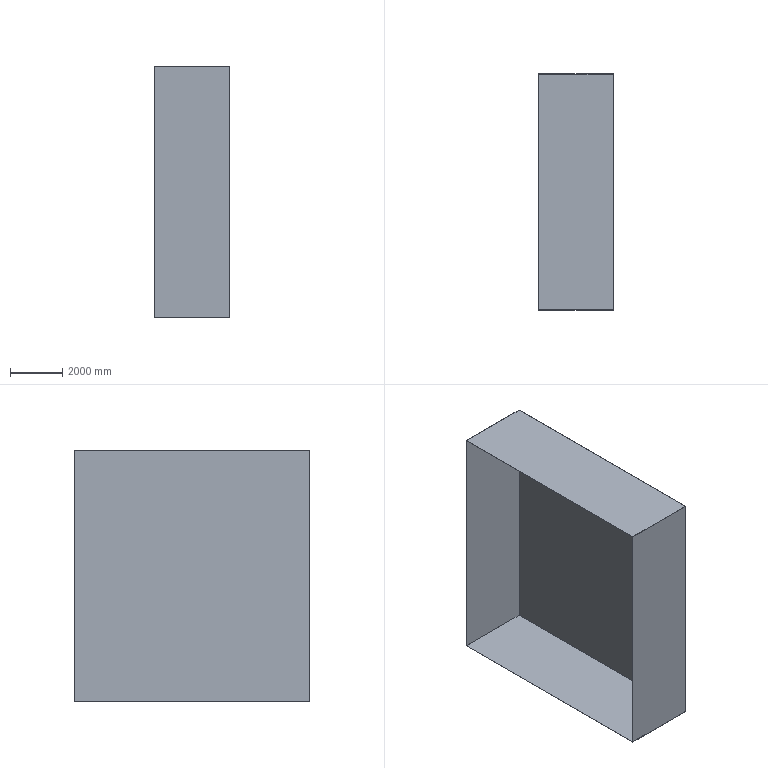Component | NX | CHUNSHUIJINCAO_BAN | 1 solid | 11 faces | box 2850 x 9000 x 9600 mm | volume 1152771264 mm3 | plane 11
STEP:
#1=CARTESIAN_POINT('',(0.,0.,0.));
#2=DIRECTION('',(0.,0.,1.));
#3=DIRECTION('',(1.,0.,0.));
#4=AXIS2_PLACEMENT_3D('',#1,#2,#3);
#5=CARTESIAN_POINT('',(2850.,250.,250.));
#6=VERTEX_POINT('',#5);
#7=CARTESIAN_POINT('',(2850.,250.,9850.));
#8=VERTEX_POINT('',#7);
#9=CARTESIAN_POINT('',(2850.,250.,250.));
#10=DIRECTION('',(0.,0.,1.));
#11=VECTOR('',#10,1.);
#12=LINE('',#9,#11);
#13=CARTESIAN_POINT('',(-0.,250.,250.));
#14=DIRECTION('',(0.,1.,0.));
#15=DIRECTION('',(1.,0.,0.));
#16=AXIS2_PLACEMENT_3D('',#13,#14,#15);
#17=PLANE('',#16);
#18=CARTESIAN_POINT('',(2850.,0.));
#19=DIRECTION('',(0.,-1.));
#20=VECTOR('',#19,1.);
#21=LINE('',#18,#20);
#22=(GEOMETRIC_REPRESENTATION_CONTEXT(2)PARAMETRIC_REPRESENTATION_CONTEXT()REPRESENTATION_CONTEXT('',''));
#23=DEFINITIONAL_REPRESENTATION('',(#21),#22);
#24=PCURVE('',#17,#23);
#25=CARTESIAN_POINT('',(2850.,250.,9850.));
#26=DIRECTION('',(-1.,0.,0.));
#27=DIRECTION('',(0.,1.,0.));
#28=AXIS2_PLACEMENT_3D('',#25,#26,#27);
#29=PLANE('',#28);
#30=CARTESIAN_POINT('',(0.,9600.));
#31=DIRECTION('',(0.,-1.));
#32=VECTOR('',#31,1.);
#33=LINE('',#30,#32);
#34=(GEOMETRIC_REPRESENTATION_CONTEXT(2)PARAMETRIC_REPRESENTATION_CONTEXT()REPRESENTATION_CONTEXT('',''));
#35=DEFINITIONAL_REPRESENTATION('',(#33),#34);
#36=PCURVE('',#29,#35);
#37=SURFACE_CURVE('',#12,(#24,#36),.PCURVE_S1.);
#38=EDGE_CURVE('',#6,#8,#37,.T.);
#39=ORIENTED_EDGE('',*,*,#38,.T.);
#40=CARTESIAN_POINT('',(-0.,250.,9850.));
#41=VERTEX_POINT('',#40);
#42=CARTESIAN_POINT('',(-0.,250.,9850.));
#43=DIRECTION('',(1.,0.,0.));
#44=VECTOR('',#43,1.);
#45=LINE('',#42,#44);
#46=CARTESIAN_POINT('',(0.,-9600.));
#47=DIRECTION('',(1.,0.));
#48=VECTOR('',#47,1.);
#49=LINE('',#46,#48);
#50=(GEOMETRIC_REPRESENTATION_CONTEXT(2)PARAMETRIC_REPRESENTATION_CONTEXT()REPRESENTATION_CONTEXT('',''));
#51=DEFINITIONAL_REPRESENTATION('',(#49),#50);
#52=PCURVE('',#17,#51);
#53=CARTESIAN_POINT('',(-0.,250.,9850.));
#54=DIRECTION('',(0.,0.,-1.));
#55=DIRECTION('',(-1.,0.,0.));
#56=AXIS2_PLACEMENT_3D('',#53,#54,#55);
#57=PLANE('',#56);
#58=CARTESIAN_POINT('',(0.,0.));
#59=DIRECTION('',(-1.,0.));
#60=VECTOR('',#59,1.);
#61=LINE('',#58,#60);
#62=(GEOMETRIC_REPRESENTATION_CONTEXT(2)PARAMETRIC_REPRESENTATION_CONTEXT()REPRESENTATION_CONTEXT('',''));
#63=DEFINITIONAL_REPRESENTATION('',(#61),#62);
#64=PCURVE('',#57,#63);
#65=SURFACE_CURVE('',#45,(#52,#64),.PCURVE_S1.);
#66=EDGE_CURVE('',#41,#8,#65,.T.);
#67=ORIENTED_EDGE('',*,*,#66,.F.);
#68=CARTESIAN_POINT('',(-0.,250.,250.));
#69=VERTEX_POINT('',#68);
#70=CARTESIAN_POINT('',(-0.,250.,250.));
#71=DIRECTION('',(0.,0.,1.));
#72=VECTOR('',#71,1.);
#73=LINE('',#70,#72);
#74=CARTESIAN_POINT('',(0.,0.));
#75=DIRECTION('',(0.,-1.));
#76=VECTOR('',#75,1.);
#77=LINE('',#74,#76);
#78=(GEOMETRIC_REPRESENTATION_CONTEXT(2)PARAMETRIC_REPRESENTATION_CONTEXT()REPRESENTATION_CONTEXT('',''));
#79=DEFINITIONAL_REPRESENTATION('',(#77),#78);
#80=PCURVE('',#17,#79);
#81=CARTESIAN_POINT('',(-0.,250.,9850.));
#82=DIRECTION('',(-1.,0.,0.));
#83=DIRECTION('',(0.,1.,0.));
#84=AXIS2_PLACEMENT_3D('',#81,#82,#83);
#85=PLANE('',#84);
#86=CARTESIAN_POINT('',(0.,9600.));
#87=DIRECTION('',(0.,-1.));
#88=VECTOR('',#87,1.);
#89=LINE('',#86,#88);
#90=(GEOMETRIC_REPRESENTATION_CONTEXT(2)PARAMETRIC_REPRESENTATION_CONTEXT()REPRESENTATION_CONTEXT('',''));
#91=DEFINITIONAL_REPRESENTATION('',(#89),#90);
#92=PCURVE('',#85,#91);
#93=SURFACE_CURVE('',#73,(#80,#92),.PCURVE_S1.);
#94=EDGE_CURVE('',#69,#41,#93,.T.);
#95=ORIENTED_EDGE('',*,*,#94,.F.);
#96=CARTESIAN_POINT('',(-0.,250.,250.));
#97=DIRECTION('',(1.,0.,0.));
#98=VECTOR('',#97,1.);
#99=LINE('',#96,#98);
#100=CARTESIAN_POINT('',(0.,0.));
#101=DIRECTION('',(1.,0.));
#102=VECTOR('',#101,1.);
#103=LINE('',#100,#102);
#104=(GEOMETRIC_REPRESENTATION_CONTEXT(2)PARAMETRIC_REPRESENTATION_CONTEXT()REPRESENTATION_CONTEXT('',''));
#105=DEFINITIONAL_REPRESENTATION('',(#103),#104);
#106=PCURVE('',#17,#105);
#107=CARTESIAN_POINT('',(-0.,9250.,250.));
#108=DIRECTION('',(0.,0.,1.));
#109=DIRECTION('',(1.,0.,0.));
#110=AXIS2_PLACEMENT_3D('',#107,#108,#109);
#111=PLANE('',#110);
#112=CARTESIAN_POINT('',(0.,-9000.));
#113=DIRECTION('',(1.,0.));
#114=VECTOR('',#113,1.);
#115=LINE('',#112,#114);
#116=(GEOMETRIC_REPRESENTATION_CONTEXT(2)PARAMETRIC_REPRESENTATION_CONTEXT()REPRESENTATION_CONTEXT('',''));
#117=DEFINITIONAL_REPRESENTATION('',(#115),#116);
#118=PCURVE('',#111,#117);
#119=SURFACE_CURVE('',#99,(#106,#118),.PCURVE_S1.);
#120=EDGE_CURVE('',#69,#6,#119,.T.);
#121=ORIENTED_EDGE('',*,*,#120,.T.);
#122=EDGE_LOOP('',(#39,#67,#95,#121));
#123=FACE_BOUND('',#122,.T.);
#124=ADVANCED_FACE('',(#123),#17,.F.);
#125=CARTESIAN_POINT('',(2850.,9250.,9850.));
#126=VERTEX_POINT('',#125);
#127=CARTESIAN_POINT('',(2850.,250.,9850.));
#128=DIRECTION('',(0.,1.,0.));
#129=VECTOR('',#128,1.);
#130=LINE('',#127,#129);
#131=CARTESIAN_POINT('',(-2850.,0.));
#132=DIRECTION('',(0.,1.));
#133=VECTOR('',#132,1.);
#134=LINE('',#131,#133);
#135=(GEOMETRIC_REPRESENTATION_CONTEXT(2)PARAMETRIC_REPRESENTATION_CONTEXT()REPRESENTATION_CONTEXT('',''));
#136=DEFINITIONAL_REPRESENTATION('',(#134),#135);
#137=PCURVE('',#57,#136);
#138=CARTESIAN_POINT('',(0.,0.));
#139=DIRECTION('',(1.,0.));
#140=VECTOR('',#139,1.);
#141=LINE('',#138,#140);
#142=(GEOMETRIC_REPRESENTATION_CONTEXT(2)PARAMETRIC_REPRESENTATION_CONTEXT()REPRESENTATION_CONTEXT('',''));
#143=DEFINITIONAL_REPRESENTATION('',(#141),#142);
#144=PCURVE('',#29,#143);
#145=SURFACE_CURVE('',#130,(#137,#144),.PCURVE_S1.);
#146=EDGE_CURVE('',#8,#126,#145,.T.);
#147=ORIENTED_EDGE('',*,*,#146,.T.);
#148=CARTESIAN_POINT('',(-0.,9250.,9850.));
#149=VERTEX_POINT('',#148);
#150=CARTESIAN_POINT('',(-0.,9250.,9850.));
#151=DIRECTION('',(1.,0.,0.));
#152=VECTOR('',#151,1.);
#153=LINE('',#150,#152);
#154=CARTESIAN_POINT('',(0.,9000.));
#155=DIRECTION('',(-1.,0.));
#156=VECTOR('',#155,1.);
#157=LINE('',#154,#156);
#158=(GEOMETRIC_REPRESENTATION_CONTEXT(2)PARAMETRIC_REPRESENTATION_CONTEXT()REPRESENTATION_CONTEXT('',''));
#159=DEFINITIONAL_REPRESENTATION('',(#157),#158);
#160=PCURVE('',#57,#159);
#161=CARTESIAN_POINT('',(-0.,9250.,9850.));
#162=DIRECTION('',(0.,-1.,0.));
#163=DIRECTION('',(-1.,0.,0.));
#164=AXIS2_PLACEMENT_3D('',#161,#162,#163);
#165=PLANE('',#164);
#166=CARTESIAN_POINT('',(0.,0.));
#167=DIRECTION('',(-1.,0.));
#168=VECTOR('',#167,1.);
#169=LINE('',#166,#168);
#170=(GEOMETRIC_REPRESENTATION_CONTEXT(2)PARAMETRIC_REPRESENTATION_CONTEXT()REPRESENTATION_CONTEXT('',''));
#171=DEFINITIONAL_REPRESENTATION('',(#169),#170);
#172=PCURVE('',#165,#171);
#173=SURFACE_CURVE('',#153,(#160,#172),.PCURVE_S1.);
#174=EDGE_CURVE('',#149,#126,#173,.T.);
#175=ORIENTED_EDGE('',*,*,#174,.F.);
#176=CARTESIAN_POINT('',(-0.,250.,9850.));
#177=DIRECTION('',(0.,1.,0.));
#178=VECTOR('',#177,1.);
#179=LINE('',#176,#178);
#180=CARTESIAN_POINT('',(0.,0.));
#181=DIRECTION('',(0.,1.));
#182=VECTOR('',#181,1.);
#183=LINE('',#180,#182);
#184=(GEOMETRIC_REPRESENTATION_CONTEXT(2)PARAMETRIC_REPRESENTATION_CONTEXT()REPRESENTATION_CONTEXT('',''));
#185=DEFINITIONAL_REPRESENTATION('',(#183),#184);
#186=PCURVE('',#57,#185);
#187=CARTESIAN_POINT('',(0.,0.));
#188=DIRECTION('',(1.,0.));
#189=VECTOR('',#188,1.);
#190=LINE('',#187,#189);
#191=(GEOMETRIC_REPRESENTATION_CONTEXT(2)PARAMETRIC_REPRESENTATION_CONTEXT()REPRESENTATION_CONTEXT('',''));
#192=DEFINITIONAL_REPRESENTATION('',(#190),#191);
#193=PCURVE('',#85,#192);
#194=SURFACE_CURVE('',#179,(#186,#193),.PCURVE_S1.);
#195=EDGE_CURVE('',#41,#149,#194,.T.);
#196=ORIENTED_EDGE('',*,*,#195,.F.);
#197=ORIENTED_EDGE('',*,*,#66,.T.);
#198=EDGE_LOOP('',(#147,#175,#196,#197));
#199=FACE_BOUND('',#198,.T.);
#200=ADVANCED_FACE('',(#199),#57,.F.);
#201=CARTESIAN_POINT('',(2850.,9250.,250.));
#202=VERTEX_POINT('',#201);
#203=CARTESIAN_POINT('',(2850.,9250.,9850.));
#204=DIRECTION('',(0.,0.,-1.));
#205=VECTOR('',#204,1.);
#206=LINE('',#203,#205);
#207=CARTESIAN_POINT('',(-2850.,0.));
#208=DIRECTION('',(0.,1.));
#209=VECTOR('',#208,1.);
#210=LINE('',#207,#209);
#211=(GEOMETRIC_REPRESENTATION_CONTEXT(2)PARAMETRIC_REPRESENTATION_CONTEXT()REPRESENTATION_CONTEXT('',''));
#212=DEFINITIONAL_REPRESENTATION('',(#210),#211);
#213=PCURVE('',#165,#212);
#214=CARTESIAN_POINT('',(9000.,0.));
#215=DIRECTION('',(0.,1.));
#216=VECTOR('',#215,1.);
#217=LINE('',#214,#216);
#218=(GEOMETRIC_REPRESENTATION_CONTEXT(2)PARAMETRIC_REPRESENTATION_CONTEXT()REPRESENTATION_CONTEXT('',''));
#219=DEFINITIONAL_REPRESENTATION('',(#217),#218);
#220=PCURVE('',#29,#219);
#221=SURFACE_CURVE('',#206,(#213,#220),.PCURVE_S1.);
#222=EDGE_CURVE('',#126,#202,#221,.T.);
#223=ORIENTED_EDGE('',*,*,#222,.T.);
#224=CARTESIAN_POINT('',(-0.,9250.,250.));
#225=VERTEX_POINT('',#224);
#226=CARTESIAN_POINT('',(-0.,9250.,250.));
#227=DIRECTION('',(1.,0.,0.));
#228=VECTOR('',#227,1.);
#229=LINE('',#226,#228);
#230=CARTESIAN_POINT('',(0.,9600.));
#231=DIRECTION('',(-1.,0.));
#232=VECTOR('',#231,1.);
#233=LINE('',#230,#232);
#234=(GEOMETRIC_REPRESENTATION_CONTEXT(2)PARAMETRIC_REPRESENTATION_CONTEXT()REPRESENTATION_CONTEXT('',''));
#235=DEFINITIONAL_REPRESENTATION('',(#233),#234);
#236=PCURVE('',#165,#235);
#237=CARTESIAN_POINT('',(0.,0.));
#238=DIRECTION('',(1.,0.));
#239=VECTOR('',#238,1.);
#240=LINE('',#237,#239);
#241=(GEOMETRIC_REPRESENTATION_CONTEXT(2)PARAMETRIC_REPRESENTATION_CONTEXT()REPRESENTATION_CONTEXT('',''));
#242=DEFINITIONAL_REPRESENTATION('',(#240),#241);
#243=PCURVE('',#111,#242);
#244=SURFACE_CURVE('',#229,(#236,#243),.PCURVE_S1.);
#245=EDGE_CURVE('',#225,#202,#244,.T.);
#246=ORIENTED_EDGE('',*,*,#245,.F.);
#247=CARTESIAN_POINT('',(-0.,9250.,9850.));
#248=DIRECTION('',(0.,0.,-1.));
#249=VECTOR('',#248,1.);
#250=LINE('',#247,#249);
#251=CARTESIAN_POINT('',(0.,0.));
#252=DIRECTION('',(0.,1.));
#253=VECTOR('',#252,1.);
#254=LINE('',#251,#253);
#255=(GEOMETRIC_REPRESENTATION_CONTEXT(2)PARAMETRIC_REPRESENTATION_CONTEXT()REPRESENTATION_CONTEXT('',''));
#256=DEFINITIONAL_REPRESENTATION('',(#254),#255);
#257=PCURVE('',#165,#256);
#258=CARTESIAN_POINT('',(9000.,0.));
#259=DIRECTION('',(0.,1.));
#260=VECTOR('',#259,1.);
#261=LINE('',#258,#260);
#262=(GEOMETRIC_REPRESENTATION_CONTEXT(2)PARAMETRIC_REPRESENTATION_CONTEXT()REPRESENTATION_CONTEXT('',''));
#263=DEFINITIONAL_REPRESENTATION('',(#261),#262);
#264=PCURVE('',#85,#263);
#265=SURFACE_CURVE('',#250,(#257,#264),.PCURVE_S1.);
#266=EDGE_CURVE('',#149,#225,#265,.T.);
#267=ORIENTED_EDGE('',*,*,#266,.F.);
#268=ORIENTED_EDGE('',*,*,#174,.T.);
#269=EDGE_LOOP('',(#223,#246,#267,#268));
#270=FACE_BOUND('',#269,.T.);
#271=ADVANCED_FACE('',(#270),#165,.F.);
#272=CARTESIAN_POINT('',(2850.,9250.,250.));
#273=DIRECTION('',(0.,-1.,0.));
#274=VECTOR('',#273,1.);
#275=LINE('',#272,#274);
#276=CARTESIAN_POINT('',(2850.,0.));
#277=DIRECTION('',(0.,-1.));
#278=VECTOR('',#277,1.);
#279=LINE('',#276,#278);
#280=(GEOMETRIC_REPRESENTATION_CONTEXT(2)PARAMETRIC_REPRESENTATION_CONTEXT()REPRESENTATION_CONTEXT('',''));
#281=DEFINITIONAL_REPRESENTATION('',(#279),#280);
#282=PCURVE('',#111,#281);
#283=CARTESIAN_POINT('',(9000.,9600.));
#284=DIRECTION('',(-1.,0.));
#285=VECTOR('',#284,1.);
#286=LINE('',#283,#285);
#287=(GEOMETRIC_REPRESENTATION_CONTEXT(2)PARAMETRIC_REPRESENTATION_CONTEXT()REPRESENTATION_CONTEXT('',''));
#288=DEFINITIONAL_REPRESENTATION('',(#286),#287);
#289=PCURVE('',#29,#288);
#290=SURFACE_CURVE('',#275,(#282,#289),.PCURVE_S1.);
#291=EDGE_CURVE('',#202,#6,#290,.T.);
#292=ORIENTED_EDGE('',*,*,#291,.T.);
#293=ORIENTED_EDGE('',*,*,#120,.F.);
#294=CARTESIAN_POINT('',(-0.,9250.,250.));
#295=DIRECTION('',(0.,-1.,0.));
#296=VECTOR('',#295,1.);
#297=LINE('',#294,#296);
#298=CARTESIAN_POINT('',(0.,0.));
#299=DIRECTION('',(0.,-1.));
#300=VECTOR('',#299,1.);
#301=LINE('',#298,#300);
#302=(GEOMETRIC_REPRESENTATION_CONTEXT(2)PARAMETRIC_REPRESENTATION_CONTEXT()REPRESENTATION_CONTEXT('',''));
#303=DEFINITIONAL_REPRESENTATION('',(#301),#302);
#304=PCURVE('',#111,#303);
#305=CARTESIAN_POINT('',(9000.,9600.));
#306=DIRECTION('',(-1.,0.));
#307=VECTOR('',#306,1.);
#308=LINE('',#305,#307);
#309=(GEOMETRIC_REPRESENTATION_CONTEXT(2)PARAMETRIC_REPRESENTATION_CONTEXT()REPRESENTATION_CONTEXT('',''));
#310=DEFINITIONAL_REPRESENTATION('',(#308),#309);
#311=PCURVE('',#85,#310);
#312=SURFACE_CURVE('',#297,(#304,#311),.PCURVE_S1.);
#313=EDGE_CURVE('',#225,#69,#312,.T.);
#314=ORIENTED_EDGE('',*,*,#313,.F.);
#315=ORIENTED_EDGE('',*,*,#245,.T.);
#316=EDGE_LOOP('',(#292,#293,#314,#315));
#317=FACE_BOUND('',#316,.T.);
#318=ADVANCED_FACE('',(#317),#111,.F.);
#319=CARTESIAN_POINT('',(-0.,256.,256.));
#320=VERTEX_POINT('',#319);
#321=CARTESIAN_POINT('',(-0.,256.,9844.));
#322=VERTEX_POINT('',#321);
#323=CARTESIAN_POINT('',(-0.,256.,250.));
#324=DIRECTION('',(0.,0.,1.));
#325=VECTOR('',#324,1.);
#326=LINE('',#323,#325);
#327=CARTESIAN_POINT('',(6.,9600.));
#328=DIRECTION('',(0.,-1.));
#329=VECTOR('',#328,1.);
#330=LINE('',#327,#329);
#331=(GEOMETRIC_REPRESENTATION_CONTEXT(2)PARAMETRIC_REPRESENTATION_CONTEXT()REPRESENTATION_CONTEXT('',''));
#332=DEFINITIONAL_REPRESENTATION('',(#330),#331);
#333=PCURVE('',#85,#332);
#334=CARTESIAN_POINT('',(-0.,256.,250.));
#335=DIRECTION('',(0.,1.,0.));
#336=DIRECTION('',(1.,0.,0.));
#337=AXIS2_PLACEMENT_3D('',#334,#335,#336);
#338=PLANE('',#337);
#339=CARTESIAN_POINT('',(0.,0.));
#340=DIRECTION('',(0.,-1.));
#341=VECTOR('',#340,1.);
#342=LINE('',#339,#341);
#343=(GEOMETRIC_REPRESENTATION_CONTEXT(2)PARAMETRIC_REPRESENTATION_CONTEXT()REPRESENTATION_CONTEXT('',''));
#344=DEFINITIONAL_REPRESENTATION('',(#342),#343);
#345=PCURVE('',#338,#344);
#346=SURFACE_CURVE('',#326,(#333,#345),.PCURVE_S1.);
#347=EDGE_CURVE('',#320,#322,#346,.T.);
#348=ORIENTED_EDGE('',*,*,#347,.F.);
#349=CARTESIAN_POINT('',(-0.,9244.,256.));
#350=VERTEX_POINT('',#349);
#351=CARTESIAN_POINT('',(-0.,9250.,256.));
#352=DIRECTION('',(0.,-1.,0.));
#353=VECTOR('',#352,1.);
#354=LINE('',#351,#353);
#355=CARTESIAN_POINT('',(9000.,9594.));
#356=DIRECTION('',(-1.,0.));
#357=VECTOR('',#356,1.);
#358=LINE('',#355,#357);
#359=(GEOMETRIC_REPRESENTATION_CONTEXT(2)PARAMETRIC_REPRESENTATION_CONTEXT()REPRESENTATION_CONTEXT('',''));
#360=DEFINITIONAL_REPRESENTATION('',(#358),#359);
#361=PCURVE('',#85,#360);
#362=CARTESIAN_POINT('',(-0.,9250.,256.));
#363=DIRECTION('',(0.,0.,1.));
#364=DIRECTION('',(1.,0.,0.));
#365=AXIS2_PLACEMENT_3D('',#362,#363,#364);
#366=PLANE('',#365);
#367=CARTESIAN_POINT('',(0.,0.));
#368=DIRECTION('',(0.,-1.));
#369=VECTOR('',#368,1.);
#370=LINE('',#367,#369);
#371=(GEOMETRIC_REPRESENTATION_CONTEXT(2)PARAMETRIC_REPRESENTATION_CONTEXT()REPRESENTATION_CONTEXT('',''));
#372=DEFINITIONAL_REPRESENTATION('',(#370),#371);
#373=PCURVE('',#366,#372);
#374=SURFACE_CURVE('',#354,(#361,#373),.PCURVE_S1.);
#375=EDGE_CURVE('',#350,#320,#374,.T.);
#376=ORIENTED_EDGE('',*,*,#375,.F.);
#377=CARTESIAN_POINT('',(-0.,9244.,9844.));
#378=VERTEX_POINT('',#377);
#379=CARTESIAN_POINT('',(-0.,9244.,9850.));
#380=DIRECTION('',(0.,0.,-1.));
#381=VECTOR('',#380,1.);
#382=LINE('',#379,#381);
#383=CARTESIAN_POINT('',(8994.,0.));
#384=DIRECTION('',(0.,1.));
#385=VECTOR('',#384,1.);
#386=LINE('',#383,#385);
#387=(GEOMETRIC_REPRESENTATION_CONTEXT(2)PARAMETRIC_REPRESENTATION_CONTEXT()REPRESENTATION_CONTEXT('',''));
#388=DEFINITIONAL_REPRESENTATION('',(#386),#387);
#389=PCURVE('',#85,#388);
#390=CARTESIAN_POINT('',(-0.,9244.,9850.));
#391=DIRECTION('',(0.,-1.,0.));
#392=DIRECTION('',(-1.,0.,0.));
#393=AXIS2_PLACEMENT_3D('',#390,#391,#392);
#394=PLANE('',#393);
#395=CARTESIAN_POINT('',(0.,0.));
#396=DIRECTION('',(0.,1.));
#397=VECTOR('',#396,1.);
#398=LINE('',#395,#397);
#399=(GEOMETRIC_REPRESENTATION_CONTEXT(2)PARAMETRIC_REPRESENTATION_CONTEXT()REPRESENTATION_CONTEXT('',''));
#400=DEFINITIONAL_REPRESENTATION('',(#398),#399);
#401=PCURVE('',#394,#400);
#402=SURFACE_CURVE('',#382,(#389,#401),.PCURVE_S1.);
#403=EDGE_CURVE('',#378,#350,#402,.T.);
#404=ORIENTED_EDGE('',*,*,#403,.F.);
#405=CARTESIAN_POINT('',(-0.,250.,9844.));
#406=DIRECTION('',(0.,1.,0.));
#407=VECTOR('',#406,1.);
#408=LINE('',#405,#407);
#409=CARTESIAN_POINT('',(0.,6.));
#410=DIRECTION('',(1.,0.));
#411=VECTOR('',#410,1.);
#412=LINE('',#409,#411);
#413=(GEOMETRIC_REPRESENTATION_CONTEXT(2)PARAMETRIC_REPRESENTATION_CONTEXT()REPRESENTATION_CONTEXT('',''));
#414=DEFINITIONAL_REPRESENTATION('',(#412),#413);
#415=PCURVE('',#85,#414);
#416=CARTESIAN_POINT('',(-0.,250.,9844.));
#417=DIRECTION('',(0.,0.,-1.));
#418=DIRECTION('',(-1.,0.,0.));
#419=AXIS2_PLACEMENT_3D('',#416,#417,#418);
#420=PLANE('',#419);
#421=CARTESIAN_POINT('',(0.,0.));
#422=DIRECTION('',(0.,1.));
#423=VECTOR('',#422,1.);
#424=LINE('',#421,#423);
#425=(GEOMETRIC_REPRESENTATION_CONTEXT(2)PARAMETRIC_REPRESENTATION_CONTEXT()REPRESENTATION_CONTEXT('',''));
#426=DEFINITIONAL_REPRESENTATION('',(#424),#425);
#427=PCURVE('',#420,#426);
#428=SURFACE_CURVE('',#408,(#415,#427),.PCURVE_S1.);
#429=EDGE_CURVE('',#322,#378,#428,.T.);
#430=ORIENTED_EDGE('',*,*,#429,.F.);
#431=EDGE_LOOP('',(#348,#376,#404,#430));
#432=FACE_BOUND('',#431,.T.);
#433=ORIENTED_EDGE('',*,*,#94,.T.);
#434=ORIENTED_EDGE('',*,*,#195,.T.);
#435=ORIENTED_EDGE('',*,*,#266,.T.);
#436=ORIENTED_EDGE('',*,*,#313,.T.);
#437=EDGE_LOOP('',(#433,#434,#435,#436));
#438=FACE_BOUND('',#437,.T.);
#439=ADVANCED_FACE('',(#432,#438),#85,.T.);
#440=ORIENTED_EDGE('',*,*,#38,.F.);
#441=ORIENTED_EDGE('',*,*,#291,.F.);
#442=ORIENTED_EDGE('',*,*,#222,.F.);
#443=ORIENTED_EDGE('',*,*,#146,.F.);
#444=EDGE_LOOP('',(#440,#441,#442,#443));
#445=FACE_BOUND('',#444,.T.);
#446=ADVANCED_FACE('',(#445),#29,.F.);
#447=CARTESIAN_POINT('',(2844.,256.,256.));
#448=VERTEX_POINT('',#447);
#449=CARTESIAN_POINT('',(2844.,256.,9844.));
#450=VERTEX_POINT('',#449);
#451=CARTESIAN_POINT('',(2844.,256.,250.));
#452=DIRECTION('',(0.,0.,1.));
#453=VECTOR('',#452,1.);
#454=LINE('',#451,#453);
#455=CARTESIAN_POINT('',(2844.,0.));
#456=DIRECTION('',(0.,-1.));
#457=VECTOR('',#456,1.);
#458=LINE('',#455,#457);
#459=(GEOMETRIC_REPRESENTATION_CONTEXT(2)PARAMETRIC_REPRESENTATION_CONTEXT()REPRESENTATION_CONTEXT('',''));
#460=DEFINITIONAL_REPRESENTATION('',(#458),#459);
#461=PCURVE('',#338,#460);
#462=CARTESIAN_POINT('',(2844.,250.,9850.));
#463=DIRECTION('',(-1.,0.,0.));
#464=DIRECTION('',(0.,1.,0.));
#465=AXIS2_PLACEMENT_3D('',#462,#463,#464);
#466=PLANE('',#465);
#467=CARTESIAN_POINT('',(6.,9600.));
#468=DIRECTION('',(0.,-1.));
#469=VECTOR('',#468,1.);
#470=LINE('',#467,#469);
#471=(GEOMETRIC_REPRESENTATION_CONTEXT(2)PARAMETRIC_REPRESENTATION_CONTEXT()REPRESENTATION_CONTEXT('',''));
#472=DEFINITIONAL_REPRESENTATION('',(#470),#471);
#473=PCURVE('',#466,#472);
#474=SURFACE_CURVE('',#454,(#461,#473),.PCURVE_S1.);
#475=EDGE_CURVE('',#448,#450,#474,.T.);
#476=ORIENTED_EDGE('',*,*,#475,.F.);
#477=CARTESIAN_POINT('',(-0.,256.,256.));
#478=DIRECTION('',(1.,0.,0.));
#479=VECTOR('',#478,1.);
#480=LINE('',#477,#479);
#481=CARTESIAN_POINT('',(0.,-6.));
#482=DIRECTION('',(1.,0.));
#483=VECTOR('',#482,1.);
#484=LINE('',#481,#483);
#485=(GEOMETRIC_REPRESENTATION_CONTEXT(2)PARAMETRIC_REPRESENTATION_CONTEXT()REPRESENTATION_CONTEXT('',''));
#486=DEFINITIONAL_REPRESENTATION('',(#484),#485);
#487=PCURVE('',#338,#486);
#488=CARTESIAN_POINT('',(0.,-8994.));
#489=DIRECTION('',(1.,0.));
#490=VECTOR('',#489,1.);
#491=LINE('',#488,#490);
#492=(GEOMETRIC_REPRESENTATION_CONTEXT(2)PARAMETRIC_REPRESENTATION_CONTEXT()REPRESENTATION_CONTEXT('',''));
#493=DEFINITIONAL_REPRESENTATION('',(#491),#492);
#494=PCURVE('',#366,#493);
#495=SURFACE_CURVE('',#480,(#487,#494),.PCURVE_S1.);
#496=EDGE_CURVE('',#320,#448,#495,.T.);
#497=ORIENTED_EDGE('',*,*,#496,.F.);
#498=ORIENTED_EDGE('',*,*,#347,.T.);
#499=CARTESIAN_POINT('',(-0.,256.,9844.));
#500=DIRECTION('',(1.,0.,0.));
#501=VECTOR('',#500,1.);
#502=LINE('',#499,#501);
#503=CARTESIAN_POINT('',(0.,-9594.));
#504=DIRECTION('',(1.,0.));
#505=VECTOR('',#504,1.);
#506=LINE('',#503,#505);
#507=(GEOMETRIC_REPRESENTATION_CONTEXT(2)PARAMETRIC_REPRESENTATION_CONTEXT()REPRESENTATION_CONTEXT('',''));
#508=DEFINITIONAL_REPRESENTATION('',(#506),#507);
#509=PCURVE('',#338,#508);
#510=CARTESIAN_POINT('',(0.,6.));
#511=DIRECTION('',(-1.,0.));
#512=VECTOR('',#511,1.);
#513=LINE('',#510,#512);
#514=(GEOMETRIC_REPRESENTATION_CONTEXT(2)PARAMETRIC_REPRESENTATION_CONTEXT()REPRESENTATION_CONTEXT('',''));
#515=DEFINITIONAL_REPRESENTATION('',(#513),#514);
#516=PCURVE('',#420,#515);
#517=SURFACE_CURVE('',#502,(#509,#516),.PCURVE_S1.);
#518=EDGE_CURVE('',#322,#450,#517,.T.);
#519=ORIENTED_EDGE('',*,*,#518,.T.);
#520=EDGE_LOOP('',(#476,#497,#498,#519));
#521=FACE_BOUND('',#520,.T.);
#522=ADVANCED_FACE('',(#521),#338,.T.);
#523=CARTESIAN_POINT('',(2844.,9244.,9844.));
#524=VERTEX_POINT('',#523);
#525=CARTESIAN_POINT('',(2844.,250.,9844.));
#526=DIRECTION('',(0.,1.,0.));
#527=VECTOR('',#526,1.);
#528=LINE('',#525,#527);
#529=CARTESIAN_POINT('',(-2844.,0.));
#530=DIRECTION('',(0.,1.));
#531=VECTOR('',#530,1.);
#532=LINE('',#529,#531);
#533=(GEOMETRIC_REPRESENTATION_CONTEXT(2)PARAMETRIC_REPRESENTATION_CONTEXT()REPRESENTATION_CONTEXT('',''));
#534=DEFINITIONAL_REPRESENTATION('',(#532),#533);
#535=PCURVE('',#420,#534);
#536=CARTESIAN_POINT('',(0.,6.));
#537=DIRECTION('',(1.,0.));
#538=VECTOR('',#537,1.);
#539=LINE('',#536,#538);
#540=(GEOMETRIC_REPRESENTATION_CONTEXT(2)PARAMETRIC_REPRESENTATION_CONTEXT()REPRESENTATION_CONTEXT('',''));
#541=DEFINITIONAL_REPRESENTATION('',(#539),#540);
#542=PCURVE('',#466,#541);
#543=SURFACE_CURVE('',#528,(#535,#542),.PCURVE_S1.);
#544=EDGE_CURVE('',#450,#524,#543,.T.);
#545=ORIENTED_EDGE('',*,*,#544,.F.);
#546=ORIENTED_EDGE('',*,*,#518,.F.);
#547=ORIENTED_EDGE('',*,*,#429,.T.);
#548=CARTESIAN_POINT('',(-0.,9244.,9844.));
#549=DIRECTION('',(1.,0.,0.));
#550=VECTOR('',#549,1.);
#551=LINE('',#548,#550);
#552=CARTESIAN_POINT('',(0.,8994.));
#553=DIRECTION('',(-1.,0.));
#554=VECTOR('',#553,1.);
#555=LINE('',#552,#554);
#556=(GEOMETRIC_REPRESENTATION_CONTEXT(2)PARAMETRIC_REPRESENTATION_CONTEXT()REPRESENTATION_CONTEXT('',''));
#557=DEFINITIONAL_REPRESENTATION('',(#555),#556);
#558=PCURVE('',#420,#557);
#559=CARTESIAN_POINT('',(0.,6.));
#560=DIRECTION('',(-1.,0.));
#561=VECTOR('',#560,1.);
#562=LINE('',#559,#561);
#563=(GEOMETRIC_REPRESENTATION_CONTEXT(2)PARAMETRIC_REPRESENTATION_CONTEXT()REPRESENTATION_CONTEXT('',''));
#564=DEFINITIONAL_REPRESENTATION('',(#562),#563);
#565=PCURVE('',#394,#564);
#566=SURFACE_CURVE('',#551,(#558,#565),.PCURVE_S1.);
#567=EDGE_CURVE('',#378,#524,#566,.T.);
#568=ORIENTED_EDGE('',*,*,#567,.T.);
#569=EDGE_LOOP('',(#545,#546,#547,#568));
#570=FACE_BOUND('',#569,.T.);
#571=ADVANCED_FACE('',(#570),#420,.T.);
#572=CARTESIAN_POINT('',(2844.,9244.,256.));
#573=VERTEX_POINT('',#572);
#574=CARTESIAN_POINT('',(2844.,9244.,9850.));
#575=DIRECTION('',(0.,0.,-1.));
#576=VECTOR('',#575,1.);
#577=LINE('',#574,#576);
#578=CARTESIAN_POINT('',(-2844.,0.));
#579=DIRECTION('',(0.,1.));
#580=VECTOR('',#579,1.);
#581=LINE('',#578,#580);
#582=(GEOMETRIC_REPRESENTATION_CONTEXT(2)PARAMETRIC_REPRESENTATION_CONTEXT()REPRESENTATION_CONTEXT('',''));
#583=DEFINITIONAL_REPRESENTATION('',(#581),#582);
#584=PCURVE('',#394,#583);
#585=CARTESIAN_POINT('',(8994.,0.));
#586=DIRECTION('',(0.,1.));
#587=VECTOR('',#586,1.);
#588=LINE('',#585,#587);
#589=(GEOMETRIC_REPRESENTATION_CONTEXT(2)PARAMETRIC_REPRESENTATION_CONTEXT()REPRESENTATION_CONTEXT('',''));
#590=DEFINITIONAL_REPRESENTATION('',(#588),#589);
#591=PCURVE('',#466,#590);
#592=SURFACE_CURVE('',#577,(#584,#591),.PCURVE_S1.);
#593=EDGE_CURVE('',#524,#573,#592,.T.);
#594=ORIENTED_EDGE('',*,*,#593,.F.);
#595=ORIENTED_EDGE('',*,*,#567,.F.);
#596=ORIENTED_EDGE('',*,*,#403,.T.);
#597=CARTESIAN_POINT('',(-0.,9244.,256.));
#598=DIRECTION('',(1.,0.,0.));
#599=VECTOR('',#598,1.);
#600=LINE('',#597,#599);
#601=CARTESIAN_POINT('',(0.,9594.));
#602=DIRECTION('',(-1.,0.));
#603=VECTOR('',#602,1.);
#604=LINE('',#601,#603);
#605=(GEOMETRIC_REPRESENTATION_CONTEXT(2)PARAMETRIC_REPRESENTATION_CONTEXT()REPRESENTATION_CONTEXT('',''));
#606=DEFINITIONAL_REPRESENTATION('',(#604),#605);
#607=PCURVE('',#394,#606);
#608=CARTESIAN_POINT('',(0.,-6.));
#609=DIRECTION('',(1.,0.));
#610=VECTOR('',#609,1.);
#611=LINE('',#608,#610);
#612=(GEOMETRIC_REPRESENTATION_CONTEXT(2)PARAMETRIC_REPRESENTATION_CONTEXT()REPRESENTATION_CONTEXT('',''));
#613=DEFINITIONAL_REPRESENTATION('',(#611),#612);
#614=PCURVE('',#366,#613);
#615=SURFACE_CURVE('',#600,(#607,#614),.PCURVE_S1.);
#616=EDGE_CURVE('',#350,#573,#615,.T.);
#617=ORIENTED_EDGE('',*,*,#616,.T.);
#618=EDGE_LOOP('',(#594,#595,#596,#617));
#619=FACE_BOUND('',#618,.T.);
#620=ADVANCED_FACE('',(#619),#394,.T.);
#621=CARTESIAN_POINT('',(2844.,9250.,256.));
#622=DIRECTION('',(0.,-1.,0.));
#623=VECTOR('',#622,1.);
#624=LINE('',#621,#623);
#625=CARTESIAN_POINT('',(2844.,0.));
#626=DIRECTION('',(0.,-1.));
#627=VECTOR('',#626,1.);
#628=LINE('',#625,#627);
#629=(GEOMETRIC_REPRESENTATION_CONTEXT(2)PARAMETRIC_REPRESENTATION_CONTEXT()REPRESENTATION_CONTEXT('',''));
#630=DEFINITIONAL_REPRESENTATION('',(#628),#629);
#631=PCURVE('',#366,#630);
#632=CARTESIAN_POINT('',(9000.,9594.));
#633=DIRECTION('',(-1.,0.));
#634=VECTOR('',#633,1.);
#635=LINE('',#632,#634);
#636=(GEOMETRIC_REPRESENTATION_CONTEXT(2)PARAMETRIC_REPRESENTATION_CONTEXT()REPRESENTATION_CONTEXT('',''));
#637=DEFINITIONAL_REPRESENTATION('',(#635),#636);
#638=PCURVE('',#466,#637);
#639=SURFACE_CURVE('',#624,(#631,#638),.PCURVE_S1.);
#640=EDGE_CURVE('',#573,#448,#639,.T.);
#641=ORIENTED_EDGE('',*,*,#640,.F.);
#642=ORIENTED_EDGE('',*,*,#616,.F.);
#643=ORIENTED_EDGE('',*,*,#375,.T.);
#644=ORIENTED_EDGE('',*,*,#496,.T.);
#645=EDGE_LOOP('',(#641,#642,#643,#644));
#646=FACE_BOUND('',#645,.T.);
#647=ADVANCED_FACE('',(#646),#366,.T.);
#648=ORIENTED_EDGE('',*,*,#475,.T.);
#649=ORIENTED_EDGE('',*,*,#544,.T.);
#650=ORIENTED_EDGE('',*,*,#593,.T.);
#651=ORIENTED_EDGE('',*,*,#640,.T.);
#652=EDGE_LOOP('',(#648,#649,#650,#651));
#653=FACE_BOUND('',#652,.T.);
#654=ADVANCED_FACE('',(#653),#466,.T.);
#655=CLOSED_SHELL('',(#124,#200,#271,#318,#439,#446,#522,#571,#620,#647,#654));
#656=MANIFOLD_SOLID_BREP('',#655);
#657=(LENGTH_UNIT()NAMED_UNIT(*)SI_UNIT(.MILLI.,.METRE.));
#658=UNCERTAINTY_MEASURE_WITH_UNIT(LENGTH_MEASURE(0.0000001),#657,'','');
#659=(NAMED_UNIT(*)PLANE_ANGLE_UNIT()SI_UNIT($,.RADIAN.));
#660=(NAMED_UNIT(*)SI_UNIT($,.STERADIAN.)SOLID_ANGLE_UNIT());
#661=(GEOMETRIC_REPRESENTATION_CONTEXT(3)GLOBAL_UNCERTAINTY_ASSIGNED_CONTEXT((#658))GLOBAL_UNIT_ASSIGNED_CONTEXT((#657,#659,#660))REPRESENTATION_CONTEXT('',''));
#662=ADVANCED_BREP_SHAPE_REPRESENTATION('',(#4,#656),#661);